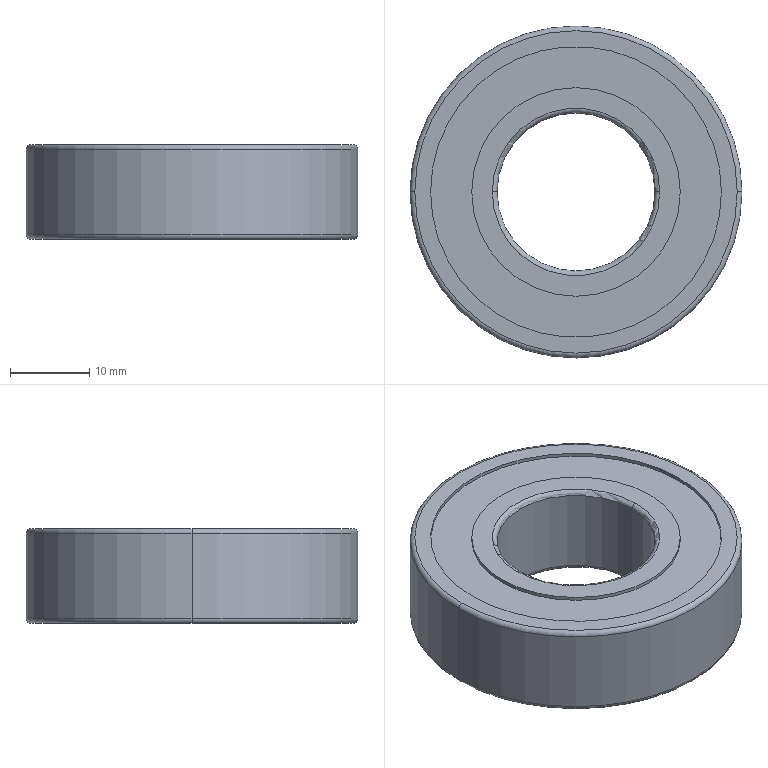Component | SolidWorks | Q1-A12-S21-Q1A.SLDASQ-1_Q1-BGSBB6004ZZ-40.sldasQ-1_Q1-bearing_6004-1 | 1 solid | 26 faces | box 42 x 42 x 12 mm | volume 12378 mm3 | cylinder 12 | torus 8 | plane 6 | commonest cylinder face diameters 26.4 x4 36.8 x4 42 x2 20 x2
build123d program:
from build123d import *


with BuildPart() as part:
    # Sketch1 → Revolve1 (revolve)
    with BuildSketch(Plane.XY, mode=Mode.PRIVATE) as revolve1_sk:
        with BuildLine():
            Line((0.6, 10), (11.4, 10))
            ThreePointArc((11.4, 10), (11.824, 10.176), (12, 10.6))
            Line((12, 10.6), (12, 13.2))
            Line((12, 13.2), (11.567, 13.2))
            Line((11.567, 13.2), (11.567, 18.4))
            Line((11.567, 18.4), (12, 18.4))
            Line((12, 18.4), (12, 20.4))
            ThreePointArc((12, 20.4), (11.824, 20.824), (11.4, 21))
            Line((11.4, 21), (0.6, 21))
            ThreePointArc((0.6, 21), (0.1757, 20.824), (0, 20.4))
            Line((0, 20.4), (0, 18.4))
            Line((0, 18.4), (0.433, 18.4))
            Line((0.433, 18.4), (0.433, 13.2))
            Line((0.433, 13.2), (0, 13.2))
            Line((0, 13.2), (0, 10.6))
            ThreePointArc((0, 10.6), (0.1757, 10.176), (0.6, 10))
        make_face()
    revolve(revolve1_sk.sketch.rotate(Axis((12, 0, 0), (-1, 0, 0)), 270), axis=Axis((12, 0, 0), (-1, 0, 0)))


solid = part.part

# Placed as in the assembly
solid = solid.moved(Location((0, 0, -137.45), (0, 90, 0)))
STEP:
#1=COLOUR_RGB('',0.7922,0.8196,0.9333);
#2=FILL_AREA_STYLE_COLOUR('',#1);
#3=FILL_AREA_STYLE('',(#2));
#4=SURFACE_STYLE_FILL_AREA(#3);
#5=SURFACE_SIDE_STYLE('',(#4));
#6=SURFACE_STYLE_USAGE(.BOTH.,#5);
#7=PRESENTATION_STYLE_ASSIGNMENT((#6));
#8=CARTESIAN_POINT('',(0.5197,0.,-5.867));
#9=VERTEX_POINT('',#8);
#10=CARTESIAN_POINT('',(-0.5197,0.,-5.867));
#11=VERTEX_POINT('',#10);
#12=CARTESIAN_POINT('',(-0.,0.,-5.867));
#13=DIRECTION('',(-0.,0.,-1.));
#14=DIRECTION('',(1.,0.,0.));
#15=AXIS2_PLACEMENT_3D('',#12,#13,#14);
#16=CIRCLE('',#15,0.5197);
#17=EDGE_CURVE('',#9,#11,#16,.T.);
#18=ORIENTED_EDGE('',*,*,#17,.T.);
#19=CARTESIAN_POINT('',(-0.5197,0.,-5.884));
#20=VERTEX_POINT('',#19);
#21=CARTESIAN_POINT('',(-0.5197,0.,-5.411));
#22=DIRECTION('',(-0.,0.,-1.));
#23=VECTOR('',#22,39.37);
#24=LINE('',#21,#23);
#25=EDGE_CURVE('',#11,#20,#24,.T.);
#26=ORIENTED_EDGE('',*,*,#25,.T.);
#27=CARTESIAN_POINT('',(0.5197,0.,-5.884));
#28=VERTEX_POINT('',#27);
#29=CARTESIAN_POINT('',(-0.,0.,-5.884));
#30=DIRECTION('',(-0.,0.,-1.));
#31=DIRECTION('',(1.,0.,0.));
#32=AXIS2_PLACEMENT_3D('',#29,#30,#31);
#33=CIRCLE('',#32,0.5197);
#34=EDGE_CURVE('',#28,#20,#33,.T.);
#35=ORIENTED_EDGE('',*,*,#34,.F.);
#36=CARTESIAN_POINT('',(0.5197,0.,-5.411));
#37=DIRECTION('',(-0.,0.,-1.));
#38=VECTOR('',#37,39.37);
#39=LINE('',#36,#38);
#40=EDGE_CURVE('',#9,#28,#39,.T.);
#41=ORIENTED_EDGE('',*,*,#40,.F.);
#42=EDGE_LOOP('',(#18,#26,#35,#41));
#43=FACE_OUTER_BOUND('',#42,.T.);
#44=CARTESIAN_POINT('',(-0.,0.,-5.411));
#45=DIRECTION('',(-0.,0.,-1.));
#46=DIRECTION('',(1.,0.,0.));
#47=AXIS2_PLACEMENT_3D('',#44,#45,#46);
#48=CYLINDRICAL_SURFACE('',#47,0.5197);
#49=ADVANCED_FACE('',(#43),#48,.T.);
#50=CARTESIAN_POINT('',(-0.7244,-0.,-5.867));
#51=VERTEX_POINT('',#50);
#52=CARTESIAN_POINT('',(0.7244,0.,-5.867));
#53=VERTEX_POINT('',#52);
#54=CARTESIAN_POINT('',(-0.,0.,-5.867));
#55=DIRECTION('',(-0.,0.,-1.));
#56=DIRECTION('',(1.,0.,0.));
#57=AXIS2_PLACEMENT_3D('',#54,#55,#56);
#58=CIRCLE('',#57,0.7244);
#59=EDGE_CURVE('',#51,#53,#58,.T.);
#60=ORIENTED_EDGE('',*,*,#59,.F.);
#61=CARTESIAN_POINT('',(-0.7244,-0.,-5.884));
#62=VERTEX_POINT('',#61);
#63=CARTESIAN_POINT('',(-0.7244,-0.,-5.411));
#64=DIRECTION('',(-0.,0.,-1.));
#65=VECTOR('',#64,39.37);
#66=LINE('',#63,#65);
#67=EDGE_CURVE('',#51,#62,#66,.T.);
#68=ORIENTED_EDGE('',*,*,#67,.T.);
#69=CARTESIAN_POINT('',(0.7244,0.,-5.884));
#70=VERTEX_POINT('',#69);
#71=CARTESIAN_POINT('',(-0.,0.,-5.884));
#72=DIRECTION('',(-0.,0.,-1.));
#73=DIRECTION('',(1.,0.,0.));
#74=AXIS2_PLACEMENT_3D('',#71,#72,#73);
#75=CIRCLE('',#74,0.7244);
#76=EDGE_CURVE('',#62,#70,#75,.T.);
#77=ORIENTED_EDGE('',*,*,#76,.T.);
#78=CARTESIAN_POINT('',(0.7244,0.,-5.411));
#79=DIRECTION('',(-0.,0.,-1.));
#80=VECTOR('',#79,39.37);
#81=LINE('',#78,#80);
#82=EDGE_CURVE('',#53,#70,#81,.T.);
#83=ORIENTED_EDGE('',*,*,#82,.F.);
#84=EDGE_LOOP('',(#60,#68,#77,#83));
#85=FACE_OUTER_BOUND('',#84,.T.);
#86=CARTESIAN_POINT('',(-0.,0.,-5.411));
#87=DIRECTION('',(-0.,0.,-1.));
#88=DIRECTION('',(1.,0.,0.));
#89=AXIS2_PLACEMENT_3D('',#86,#87,#88);
#90=CYLINDRICAL_SURFACE('',#89,0.7244);
#91=ADVANCED_FACE('',(#85),#90,.F.);
#92=CARTESIAN_POINT('',(0.8268,0.,-5.86));
#93=VERTEX_POINT('',#92);
#94=CARTESIAN_POINT('',(-0.8268,-0.,-5.86));
#95=VERTEX_POINT('',#94);
#96=CARTESIAN_POINT('',(-0.,0.,-5.86));
#97=DIRECTION('',(-0.,0.,-1.));
#98=DIRECTION('',(1.,0.,0.));
#99=AXIS2_PLACEMENT_3D('',#96,#97,#98);
#100=CIRCLE('',#99,0.8268);
#101=EDGE_CURVE('',#93,#95,#100,.T.);
#102=ORIENTED_EDGE('',*,*,#101,.T.);
#103=CARTESIAN_POINT('',(-0.8031,-0.,-5.884));
#104=VERTEX_POINT('',#103);
#105=CARTESIAN_POINT('',(-0.8031,-0.,-5.86));
#106=DIRECTION('',(0.,-1.,-0.));
#107=DIRECTION('',(1.,0.,0.));
#108=AXIS2_PLACEMENT_3D('',#105,#106,#107);
#109=CIRCLE('',#108,0.02362);
#110=EDGE_CURVE('',#95,#104,#109,.T.);
#111=ORIENTED_EDGE('',*,*,#110,.T.);
#112=CARTESIAN_POINT('',(0.8031,0.,-5.884));
#113=VERTEX_POINT('',#112);
#114=CARTESIAN_POINT('',(-0.,0.,-5.884));
#115=DIRECTION('',(-0.,0.,-1.));
#116=DIRECTION('',(1.,0.,0.));
#117=AXIS2_PLACEMENT_3D('',#114,#115,#116);
#118=CIRCLE('',#117,0.8031);
#119=EDGE_CURVE('',#113,#104,#118,.T.);
#120=ORIENTED_EDGE('',*,*,#119,.F.);
#121=CARTESIAN_POINT('',(0.8031,0.,-5.86));
#122=DIRECTION('',(-0.,1.,0.));
#123=DIRECTION('',(-1.,-0.,0.));
#124=AXIS2_PLACEMENT_3D('',#121,#122,#123);
#125=CIRCLE('',#124,0.02362);
#126=EDGE_CURVE('',#93,#113,#125,.T.);
#127=ORIENTED_EDGE('',*,*,#126,.F.);
#128=EDGE_LOOP('',(#102,#111,#120,#127));
#129=FACE_OUTER_BOUND('',#128,.T.);
#130=CARTESIAN_POINT('',(-0.,0.,-5.86));
#131=DIRECTION('',(-0.,0.,-1.));
#132=DIRECTION('',(1.,0.,-0.));
#133=AXIS2_PLACEMENT_3D('',#130,#131,#132);
#134=TOROIDAL_SURFACE('',#133,0.8031,0.02362);
#135=ADVANCED_FACE('',(#129),#134,.T.);
#136=CARTESIAN_POINT('',(0.8268,0.,-5.435));
#137=VERTEX_POINT('',#136);
#138=CARTESIAN_POINT('',(-0.8268,-0.,-5.435));
#139=VERTEX_POINT('',#138);
#140=CARTESIAN_POINT('',(-0.,0.,-5.435));
#141=DIRECTION('',(-0.,0.,-1.));
#142=DIRECTION('',(1.,0.,0.));
#143=AXIS2_PLACEMENT_3D('',#140,#141,#142);
#144=CIRCLE('',#143,0.8268);
#145=EDGE_CURVE('',#137,#139,#144,.T.);
#146=ORIENTED_EDGE('',*,*,#145,.T.);
#147=CARTESIAN_POINT('',(-0.8268,-0.,-5.411));
#148=DIRECTION('',(-0.,0.,-1.));
#149=VECTOR('',#148,39.37);
#150=LINE('',#147,#149);
#151=EDGE_CURVE('',#139,#95,#150,.T.);
#152=ORIENTED_EDGE('',*,*,#151,.T.);
#153=ORIENTED_EDGE('',*,*,#101,.F.);
#154=CARTESIAN_POINT('',(0.8268,0.,-5.411));
#155=DIRECTION('',(-0.,0.,-1.));
#156=VECTOR('',#155,39.37);
#157=LINE('',#154,#156);
#158=EDGE_CURVE('',#137,#93,#157,.T.);
#159=ORIENTED_EDGE('',*,*,#158,.F.);
#160=EDGE_LOOP('',(#146,#152,#153,#159));
#161=FACE_OUTER_BOUND('',#160,.T.);
#162=CARTESIAN_POINT('',(-0.,0.,-5.411));
#163=DIRECTION('',(-0.,0.,-1.));
#164=DIRECTION('',(1.,0.,0.));
#165=AXIS2_PLACEMENT_3D('',#162,#163,#164);
#166=CYLINDRICAL_SURFACE('',#165,0.8268);
#167=ADVANCED_FACE('',(#161),#166,.T.);
#168=CARTESIAN_POINT('',(0.8031,0.,-5.411));
#169=VERTEX_POINT('',#168);
#170=CARTESIAN_POINT('',(-0.8031,-0.,-5.411));
#171=VERTEX_POINT('',#170);
#172=CARTESIAN_POINT('',(-0.,0.,-5.411));
#173=DIRECTION('',(-0.,0.,-1.));
#174=DIRECTION('',(1.,0.,0.));
#175=AXIS2_PLACEMENT_3D('',#172,#173,#174);
#176=CIRCLE('',#175,0.8031);
#177=EDGE_CURVE('',#169,#171,#176,.T.);
#178=ORIENTED_EDGE('',*,*,#177,.T.);
#179=CARTESIAN_POINT('',(-0.8031,-0.,-5.435));
#180=DIRECTION('',(0.,-1.,-0.));
#181=DIRECTION('',(1.,0.,0.));
#182=AXIS2_PLACEMENT_3D('',#179,#180,#181);
#183=CIRCLE('',#182,0.02362);
#184=EDGE_CURVE('',#171,#139,#183,.T.);
#185=ORIENTED_EDGE('',*,*,#184,.T.);
#186=ORIENTED_EDGE('',*,*,#145,.F.);
#187=CARTESIAN_POINT('',(0.8031,0.,-5.435));
#188=DIRECTION('',(-0.,1.,0.));
#189=DIRECTION('',(-1.,-0.,0.));
#190=AXIS2_PLACEMENT_3D('',#187,#188,#189);
#191=CIRCLE('',#190,0.02362);
#192=EDGE_CURVE('',#169,#137,#191,.T.);
#193=ORIENTED_EDGE('',*,*,#192,.F.);
#194=EDGE_LOOP('',(#178,#185,#186,#193));
#195=FACE_OUTER_BOUND('',#194,.T.);
#196=CARTESIAN_POINT('',(-0.,0.,-5.435));
#197=DIRECTION('',(-0.,0.,-1.));
#198=DIRECTION('',(1.,0.,-0.));
#199=AXIS2_PLACEMENT_3D('',#196,#197,#198);
#200=TOROIDAL_SURFACE('',#199,0.8031,0.02362);
#201=ADVANCED_FACE('',(#195),#200,.T.);
#202=CARTESIAN_POINT('',(-0.7244,-0.,-5.411));
#203=VERTEX_POINT('',#202);
#204=CARTESIAN_POINT('',(0.7244,0.,-5.411));
#205=VERTEX_POINT('',#204);
#206=CARTESIAN_POINT('',(-0.,0.,-5.411));
#207=DIRECTION('',(-0.,0.,-1.));
#208=DIRECTION('',(1.,0.,0.));
#209=AXIS2_PLACEMENT_3D('',#206,#207,#208);
#210=CIRCLE('',#209,0.7244);
#211=EDGE_CURVE('',#203,#205,#210,.T.);
#212=ORIENTED_EDGE('',*,*,#211,.F.);
#213=CARTESIAN_POINT('',(-0.7244,-0.,-5.428));
#214=VERTEX_POINT('',#213);
#215=CARTESIAN_POINT('',(-0.7244,-0.,-5.411));
#216=DIRECTION('',(-0.,0.,-1.));
#217=VECTOR('',#216,39.37);
#218=LINE('',#215,#217);
#219=EDGE_CURVE('',#203,#214,#218,.T.);
#220=ORIENTED_EDGE('',*,*,#219,.T.);
#221=CARTESIAN_POINT('',(0.7244,0.,-5.428));
#222=VERTEX_POINT('',#221);
#223=CARTESIAN_POINT('',(-0.,0.,-5.428));
#224=DIRECTION('',(-0.,0.,-1.));
#225=DIRECTION('',(1.,0.,0.));
#226=AXIS2_PLACEMENT_3D('',#223,#224,#225);
#227=CIRCLE('',#226,0.7244);
#228=EDGE_CURVE('',#214,#222,#227,.T.);
#229=ORIENTED_EDGE('',*,*,#228,.T.);
#230=CARTESIAN_POINT('',(0.7244,0.,-5.411));
#231=DIRECTION('',(-0.,0.,-1.));
#232=VECTOR('',#231,39.37);
#233=LINE('',#230,#232);
#234=EDGE_CURVE('',#205,#222,#233,.T.);
#235=ORIENTED_EDGE('',*,*,#234,.F.);
#236=EDGE_LOOP('',(#212,#220,#229,#235));
#237=FACE_OUTER_BOUND('',#236,.T.);
#238=CARTESIAN_POINT('',(-0.,0.,-5.411));
#239=DIRECTION('',(-0.,0.,-1.));
#240=DIRECTION('',(1.,0.,0.));
#241=AXIS2_PLACEMENT_3D('',#238,#239,#240);
#242=CYLINDRICAL_SURFACE('',#241,0.7244);
#243=ADVANCED_FACE('',(#237),#242,.F.);
#244=CARTESIAN_POINT('',(0.5197,0.,-5.411));
#245=VERTEX_POINT('',#244);
#246=CARTESIAN_POINT('',(-0.5197,0.,-5.411));
#247=VERTEX_POINT('',#246);
#248=CARTESIAN_POINT('',(-0.,0.,-5.411));
#249=DIRECTION('',(-0.,0.,-1.));
#250=DIRECTION('',(1.,0.,0.));
#251=AXIS2_PLACEMENT_3D('',#248,#249,#250);
#252=CIRCLE('',#251,0.5197);
#253=EDGE_CURVE('',#245,#247,#252,.T.);
#254=ORIENTED_EDGE('',*,*,#253,.T.);
#255=CARTESIAN_POINT('',(-0.5197,0.,-5.428));
#256=VERTEX_POINT('',#255);
#257=CARTESIAN_POINT('',(-0.5197,0.,-5.411));
#258=DIRECTION('',(-0.,0.,-1.));
#259=VECTOR('',#258,39.37);
#260=LINE('',#257,#259);
#261=EDGE_CURVE('',#247,#256,#260,.T.);
#262=ORIENTED_EDGE('',*,*,#261,.T.);
#263=CARTESIAN_POINT('',(0.5197,0.,-5.428));
#264=VERTEX_POINT('',#263);
#265=CARTESIAN_POINT('',(-0.,0.,-5.428));
#266=DIRECTION('',(-0.,0.,-1.));
#267=DIRECTION('',(1.,0.,0.));
#268=AXIS2_PLACEMENT_3D('',#265,#266,#267);
#269=CIRCLE('',#268,0.5197);
#270=EDGE_CURVE('',#264,#256,#269,.T.);
#271=ORIENTED_EDGE('',*,*,#270,.F.);
#272=CARTESIAN_POINT('',(0.5197,0.,-5.411));
#273=DIRECTION('',(-0.,0.,-1.));
#274=VECTOR('',#273,39.37);
#275=LINE('',#272,#274);
#276=EDGE_CURVE('',#245,#264,#275,.T.);
#277=ORIENTED_EDGE('',*,*,#276,.F.);
#278=EDGE_LOOP('',(#254,#262,#271,#277));
#279=FACE_OUTER_BOUND('',#278,.T.);
#280=CARTESIAN_POINT('',(-0.,0.,-5.411));
#281=DIRECTION('',(-0.,0.,-1.));
#282=DIRECTION('',(1.,0.,0.));
#283=AXIS2_PLACEMENT_3D('',#280,#281,#282);
#284=CYLINDRICAL_SURFACE('',#283,0.5197);
#285=ADVANCED_FACE('',(#279),#284,.T.);
#286=CARTESIAN_POINT('',(0.3937,0.,-5.435));
#287=VERTEX_POINT('',#286);
#288=CARTESIAN_POINT('',(-0.3937,0.,-5.435));
#289=VERTEX_POINT('',#288);
#290=CARTESIAN_POINT('',(-0.,0.,-5.435));
#291=DIRECTION('',(-0.,0.,-1.));
#292=DIRECTION('',(1.,0.,0.));
#293=AXIS2_PLACEMENT_3D('',#290,#291,#292);
#294=CIRCLE('',#293,0.3937);
#295=EDGE_CURVE('',#287,#289,#294,.T.);
#296=ORIENTED_EDGE('',*,*,#295,.T.);
#297=CARTESIAN_POINT('',(-0.4173,0.,-5.411));
#298=VERTEX_POINT('',#297);
#299=CARTESIAN_POINT('',(-0.4173,0.,-5.435));
#300=DIRECTION('',(0.,-1.,-0.));
#301=DIRECTION('',(1.,0.,0.));
#302=AXIS2_PLACEMENT_3D('',#299,#300,#301);
#303=CIRCLE('',#302,0.02362);
#304=EDGE_CURVE('',#289,#298,#303,.T.);
#305=ORIENTED_EDGE('',*,*,#304,.T.);
#306=CARTESIAN_POINT('',(0.4173,0.,-5.411));
#307=VERTEX_POINT('',#306);
#308=CARTESIAN_POINT('',(-0.,0.,-5.411));
#309=DIRECTION('',(-0.,0.,-1.));
#310=DIRECTION('',(1.,0.,0.));
#311=AXIS2_PLACEMENT_3D('',#308,#309,#310);
#312=CIRCLE('',#311,0.4173);
#313=EDGE_CURVE('',#307,#298,#312,.T.);
#314=ORIENTED_EDGE('',*,*,#313,.F.);
#315=CARTESIAN_POINT('',(0.4173,0.,-5.435));
#316=DIRECTION('',(-0.,1.,0.));
#317=DIRECTION('',(-1.,-0.,0.));
#318=AXIS2_PLACEMENT_3D('',#315,#316,#317);
#319=CIRCLE('',#318,0.02362);
#320=EDGE_CURVE('',#287,#307,#319,.T.);
#321=ORIENTED_EDGE('',*,*,#320,.F.);
#322=EDGE_LOOP('',(#296,#305,#314,#321));
#323=FACE_OUTER_BOUND('',#322,.T.);
#324=CARTESIAN_POINT('',(-0.,0.,-5.435));
#325=DIRECTION('',(-0.,0.,-1.));
#326=DIRECTION('',(1.,0.,-0.));
#327=AXIS2_PLACEMENT_3D('',#324,#325,#326);
#328=TOROIDAL_SURFACE('',#327,0.4173,0.02362);
#329=ADVANCED_FACE('',(#323),#328,.T.);
#330=CARTESIAN_POINT('',(-0.,0.,-5.435));
#331=DIRECTION('',(-0.,0.,-1.));
#332=DIRECTION('',(1.,0.,0.));
#333=AXIS2_PLACEMENT_3D('',#330,#331,#332);
#334=CIRCLE('',#333,0.3937);
#335=EDGE_CURVE('',#289,#287,#334,.T.);
#336=ORIENTED_EDGE('',*,*,#335,.F.);
#337=CARTESIAN_POINT('',(-0.3937,0.,-5.86));
#338=VERTEX_POINT('',#337);
#339=CARTESIAN_POINT('',(-0.3937,0.,-5.411));
#340=DIRECTION('',(-0.,0.,-1.));
#341=VECTOR('',#340,39.37);
#342=LINE('',#339,#341);
#343=EDGE_CURVE('',#289,#338,#342,.T.);
#344=ORIENTED_EDGE('',*,*,#343,.T.);
#345=CARTESIAN_POINT('',(0.3937,0.,-5.86));
#346=VERTEX_POINT('',#345);
#347=CARTESIAN_POINT('',(-0.,0.,-5.86));
#348=DIRECTION('',(-0.,0.,-1.));
#349=DIRECTION('',(1.,0.,0.));
#350=AXIS2_PLACEMENT_3D('',#347,#348,#349);
#351=CIRCLE('',#350,0.3937);
#352=EDGE_CURVE('',#338,#346,#351,.T.);
#353=ORIENTED_EDGE('',*,*,#352,.T.);
#354=CARTESIAN_POINT('',(0.3937,0.,-5.411));
#355=DIRECTION('',(-0.,0.,-1.));
#356=VECTOR('',#355,39.37);
#357=LINE('',#354,#356);
#358=EDGE_CURVE('',#287,#346,#357,.T.);
#359=ORIENTED_EDGE('',*,*,#358,.F.);
#360=EDGE_LOOP('',(#336,#344,#353,#359));
#361=FACE_OUTER_BOUND('',#360,.T.);
#362=CARTESIAN_POINT('',(-0.,0.,-5.411));
#363=DIRECTION('',(-0.,0.,-1.));
#364=DIRECTION('',(1.,0.,0.));
#365=AXIS2_PLACEMENT_3D('',#362,#363,#364);
#366=CYLINDRICAL_SURFACE('',#365,0.3937);
#367=ADVANCED_FACE('',(#361),#366,.F.);
#368=CARTESIAN_POINT('',(0.4173,0.,-5.884));
#369=VERTEX_POINT('',#368);
#370=CARTESIAN_POINT('',(-0.4173,0.,-5.884));
#371=VERTEX_POINT('',#370);
#372=CARTESIAN_POINT('',(-0.,0.,-5.884));
#373=DIRECTION('',(-0.,0.,-1.));
#374=DIRECTION('',(1.,0.,0.));
#375=AXIS2_PLACEMENT_3D('',#372,#373,#374);
#376=CIRCLE('',#375,0.4173);
#377=EDGE_CURVE('',#369,#371,#376,.T.);
#378=ORIENTED_EDGE('',*,*,#377,.T.);
#379=CARTESIAN_POINT('',(-0.4173,0.,-5.86));
#380=DIRECTION('',(0.,-1.,-0.));
#381=DIRECTION('',(1.,0.,0.));
#382=AXIS2_PLACEMENT_3D('',#379,#380,#381);
#383=CIRCLE('',#382,0.02362);
#384=EDGE_CURVE('',#371,#338,#383,.T.);
#385=ORIENTED_EDGE('',*,*,#384,.T.);
#386=CARTESIAN_POINT('',(-0.,0.,-5.86));
#387=DIRECTION('',(-0.,0.,-1.));
#388=DIRECTION('',(1.,0.,0.));
#389=AXIS2_PLACEMENT_3D('',#386,#387,#388);
#390=CIRCLE('',#389,0.3937);
#391=EDGE_CURVE('',#346,#338,#390,.T.);
#392=ORIENTED_EDGE('',*,*,#391,.F.);
#393=CARTESIAN_POINT('',(0.4173,0.,-5.86));
#394=DIRECTION('',(-0.,1.,0.));
#395=DIRECTION('',(-1.,-0.,0.));
#396=AXIS2_PLACEMENT_3D('',#393,#394,#395);
#397=CIRCLE('',#396,0.02362);
#398=EDGE_CURVE('',#369,#346,#397,.T.);
#399=ORIENTED_EDGE('',*,*,#398,.F.);
#400=EDGE_LOOP('',(#378,#385,#392,#399));
#401=FACE_OUTER_BOUND('',#400,.T.);
#402=CARTESIAN_POINT('',(-0.,0.,-5.86));
#403=DIRECTION('',(-0.,0.,-1.));
#404=DIRECTION('',(1.,0.,-0.));
#405=AXIS2_PLACEMENT_3D('',#402,#403,#404);
#406=TOROIDAL_SURFACE('',#405,0.4173,0.02362);
#407=ADVANCED_FACE('',(#401),#406,.T.);
#408=ORIENTED_EDGE('',*,*,#384,.F.);
#409=CARTESIAN_POINT('',(-0.,0.,-5.884));
#410=DIRECTION('',(-0.,0.,-1.));
#411=DIRECTION('',(1.,0.,0.));
#412=AXIS2_PLACEMENT_3D('',#409,#410,#411);
#413=CIRCLE('',#412,0.4173);
#414=EDGE_CURVE('',#371,#369,#413,.T.);
#415=ORIENTED_EDGE('',*,*,#414,.T.);
#416=ORIENTED_EDGE('',*,*,#398,.T.);
#417=ORIENTED_EDGE('',*,*,#352,.F.);
#418=EDGE_LOOP('',(#408,#415,#416,#417));
#419=FACE_OUTER_BOUND('',#418,.T.);
#420=CARTESIAN_POINT('',(-0.,0.,-5.86));
#421=DIRECTION('',(-0.,0.,-1.));
#422=DIRECTION('',(1.,0.,-0.));
#423=AXIS2_PLACEMENT_3D('',#420,#421,#422);
#424=TOROIDAL_SURFACE('',#423,0.4173,0.02362);
#425=ADVANCED_FACE('',(#419),#424,.T.);
#426=ORIENTED_EDGE('',*,*,#343,.F.);
#427=ORIENTED_EDGE('',*,*,#295,.F.);
#428=ORIENTED_EDGE('',*,*,#358,.T.);
#429=ORIENTED_EDGE('',*,*,#391,.T.);
#430=EDGE_LOOP('',(#426,#427,#428,#429));
#431=FACE_OUTER_BOUND('',#430,.T.);
#432=CARTESIAN_POINT('',(-0.,0.,-5.411));
#433=DIRECTION('',(-0.,0.,-1.));
#434=DIRECTION('',(1.,0.,0.));
#435=AXIS2_PLACEMENT_3D('',#432,#433,#434);
#436=CYLINDRICAL_SURFACE('',#435,0.3937);
#437=ADVANCED_FACE('',(#431),#436,.F.);
#438=ORIENTED_EDGE('',*,*,#304,.F.);
#439=ORIENTED_EDGE('',*,*,#335,.T.);
#440=ORIENTED_EDGE('',*,*,#320,.T.);
#441=CARTESIAN_POINT('',(-0.,0.,-5.411));
#442=DIRECTION('',(-0.,0.,-1.));
#443=DIRECTION('',(1.,0.,0.));
#444=AXIS2_PLACEMENT_3D('',#441,#442,#443);
#445=CIRCLE('',#444,0.4173);
#446=EDGE_CURVE('',#298,#307,#445,.T.);
#447=ORIENTED_EDGE('',*,*,#446,.F.);
#448=EDGE_LOOP('',(#438,#439,#440,#447));
#449=FACE_OUTER_BOUND('',#448,.T.);
#450=CARTESIAN_POINT('',(-0.,0.,-5.435));
#451=DIRECTION('',(-0.,0.,-1.));
#452=DIRECTION('',(1.,0.,-0.));
#453=AXIS2_PLACEMENT_3D('',#450,#451,#452);
#454=TOROIDAL_SURFACE('',#453,0.4173,0.02362);
#455=ADVANCED_FACE('',(#449),#454,.T.);
#456=ORIENTED_EDGE('',*,*,#253,.F.);
#457=CARTESIAN_POINT('',(-0.,0.,-5.411));
#458=DIRECTION('',(-0.,0.,-1.));
#459=DIRECTION('',(1.,0.,0.));
#460=AXIS2_PLACEMENT_3D('',#457,#458,#459);
#461=CIRCLE('',#460,0.5197);
#462=EDGE_CURVE('',#247,#245,#461,.T.);
#463=ORIENTED_EDGE('',*,*,#462,.F.);
#464=EDGE_LOOP('',(#456,#463));
#465=FACE_OUTER_BOUND('',#464,.T.);
#466=ORIENTED_EDGE('',*,*,#313,.T.);
#467=ORIENTED_EDGE('',*,*,#446,.T.);
#468=EDGE_LOOP('',(#466,#467));
#469=FACE_BOUND('',#468,.T.);
#470=CARTESIAN_POINT('',(-0.,-0.4173,-5.411));
#471=DIRECTION('',(0.,0.,-1.));
#472=DIRECTION('',(1.,0.,0.));
#473=AXIS2_PLACEMENT_3D('',#470,#471,#472);
#474=PLANE('',#473);
#475=ADVANCED_FACE('',(#465,#469),#474,.F.);
#476=ORIENTED_EDGE('',*,*,#261,.F.);
#477=ORIENTED_EDGE('',*,*,#462,.T.);
#478=ORIENTED_EDGE('',*,*,#276,.T.);
#479=CARTESIAN_POINT('',(-0.,0.,-5.428));
#480=DIRECTION('',(-0.,0.,-1.));
#481=DIRECTION('',(1.,0.,0.));
#482=AXIS2_PLACEMENT_3D('',#479,#480,#481);
#483=CIRCLE('',#482,0.5197);
#484=EDGE_CURVE('',#256,#264,#483,.T.);
#485=ORIENTED_EDGE('',*,*,#484,.F.);
#486=EDGE_LOOP('',(#476,#477,#478,#485));
#487=FACE_OUTER_BOUND('',#486,.T.);
#488=CARTESIAN_POINT('',(-0.,0.,-5.411));
#489=DIRECTION('',(-0.,0.,-1.));
#490=DIRECTION('',(1.,0.,0.));
#491=AXIS2_PLACEMENT_3D('',#488,#489,#490);
#492=CYLINDRICAL_SURFACE('',#491,0.5197);
#493=ADVANCED_FACE('',(#487),#492,.T.);
#494=CARTESIAN_POINT('',(-0.,0.,-5.428));
#495=DIRECTION('',(-0.,0.,-1.));
#496=DIRECTION('',(1.,0.,0.));
#497=AXIS2_PLACEMENT_3D('',#494,#495,#496);
#498=CIRCLE('',#497,0.7244);
#499=EDGE_CURVE('',#222,#214,#498,.T.);
#500=ORIENTED_EDGE('',*,*,#499,.F.);
#501=ORIENTED_EDGE('',*,*,#228,.F.);
#502=EDGE_LOOP('',(#500,#501));
#503=FACE_OUTER_BOUND('',#502,.T.);
#504=ORIENTED_EDGE('',*,*,#270,.T.);
#505=ORIENTED_EDGE('',*,*,#484,.T.);
#506=EDGE_LOOP('',(#504,#505));
#507=FACE_BOUND('',#506,.T.);
#508=CARTESIAN_POINT('',(-0.,-0.5197,-5.428));
#509=DIRECTION('',(0.,0.,-1.));
#510=DIRECTION('',(1.,0.,0.));
#511=AXIS2_PLACEMENT_3D('',#508,#509,#510);
#512=PLANE('',#511);
#513=ADVANCED_FACE('',(#503,#507),#512,.F.);
#514=ORIENTED_EDGE('',*,*,#219,.F.);
#515=CARTESIAN_POINT('',(-0.,0.,-5.411));
#516=DIRECTION('',(-0.,0.,-1.));
#517=DIRECTION('',(1.,0.,0.));
#518=AXIS2_PLACEMENT_3D('',#515,#516,#517);
#519=CIRCLE('',#518,0.7244);
#520=EDGE_CURVE('',#205,#203,#519,.T.);
#521=ORIENTED_EDGE('',*,*,#520,.F.);
#522=ORIENTED_EDGE('',*,*,#234,.T.);
#523=ORIENTED_EDGE('',*,*,#499,.T.);
#524=EDGE_LOOP('',(#514,#521,#522,#523));
#525=FACE_OUTER_BOUND('',#524,.T.);
#526=CARTESIAN_POINT('',(-0.,0.,-5.411));
#527=DIRECTION('',(-0.,0.,-1.));
#528=DIRECTION('',(1.,0.,0.));
#529=AXIS2_PLACEMENT_3D('',#526,#527,#528);
#530=CYLINDRICAL_SURFACE('',#529,0.7244);
#531=ADVANCED_FACE('',(#525),#530,.F.);
#532=ORIENTED_EDGE('',*,*,#177,.F.);
#533=CARTESIAN_POINT('',(-0.,0.,-5.411));
#534=DIRECTION('',(-0.,0.,-1.));
#535=DIRECTION('',(1.,0.,0.));
#536=AXIS2_PLACEMENT_3D('',#533,#534,#535);
#537=CIRCLE('',#536,0.8031);
#538=EDGE_CURVE('',#171,#169,#537,.T.);
#539=ORIENTED_EDGE('',*,*,#538,.F.);
#540=EDGE_LOOP('',(#532,#539));
#541=FACE_OUTER_BOUND('',#540,.T.);
#542=ORIENTED_EDGE('',*,*,#520,.T.);
#543=ORIENTED_EDGE('',*,*,#211,.T.);
#544=EDGE_LOOP('',(#542,#543));
#545=FACE_BOUND('',#544,.T.);
#546=CARTESIAN_POINT('',(-0.,-0.7244,-5.411));
#547=DIRECTION('',(0.,0.,-1.));
#548=DIRECTION('',(1.,0.,0.));
#549=AXIS2_PLACEMENT_3D('',#546,#547,#548);
#550=PLANE('',#549);
#551=ADVANCED_FACE('',(#541,#545),#550,.F.);
#552=ORIENTED_EDGE('',*,*,#184,.F.);
#553=ORIENTED_EDGE('',*,*,#538,.T.);
#554=ORIENTED_EDGE('',*,*,#192,.T.);
#555=CARTESIAN_POINT('',(-0.,0.,-5.435));
#556=DIRECTION('',(-0.,0.,-1.));
#557=DIRECTION('',(1.,0.,0.));
#558=AXIS2_PLACEMENT_3D('',#555,#556,#557);
#559=CIRCLE('',#558,0.8268);
#560=EDGE_CURVE('',#139,#137,#559,.T.);
#561=ORIENTED_EDGE('',*,*,#560,.F.);
#562=EDGE_LOOP('',(#552,#553,#554,#561));
#563=FACE_OUTER_BOUND('',#562,.T.);
#564=CARTESIAN_POINT('',(-0.,0.,-5.435));
#565=DIRECTION('',(-0.,0.,-1.));
#566=DIRECTION('',(1.,0.,-0.));
#567=AXIS2_PLACEMENT_3D('',#564,#565,#566);
#568=TOROIDAL_SURFACE('',#567,0.8031,0.02362);
#569=ADVANCED_FACE('',(#563),#568,.T.);
#570=ORIENTED_EDGE('',*,*,#151,.F.);
#571=ORIENTED_EDGE('',*,*,#560,.T.);
#572=ORIENTED_EDGE('',*,*,#158,.T.);
#573=CARTESIAN_POINT('',(-0.,0.,-5.86));
#574=DIRECTION('',(-0.,0.,-1.));
#575=DIRECTION('',(1.,0.,0.));
#576=AXIS2_PLACEMENT_3D('',#573,#574,#575);
#577=CIRCLE('',#576,0.8268);
#578=EDGE_CURVE('',#95,#93,#577,.T.);
#579=ORIENTED_EDGE('',*,*,#578,.F.);
#580=EDGE_LOOP('',(#570,#571,#572,#579));
#581=FACE_OUTER_BOUND('',#580,.T.);
#582=CARTESIAN_POINT('',(-0.,0.,-5.411));
#583=DIRECTION('',(-0.,0.,-1.));
#584=DIRECTION('',(1.,0.,0.));
#585=AXIS2_PLACEMENT_3D('',#582,#583,#584);
#586=CYLINDRICAL_SURFACE('',#585,0.8268);
#587=ADVANCED_FACE('',(#581),#586,.T.);
#588=ORIENTED_EDGE('',*,*,#110,.F.);
#589=ORIENTED_EDGE('',*,*,#578,.T.);
#590=ORIENTED_EDGE('',*,*,#126,.T.);
#591=CARTESIAN_POINT('',(-0.,0.,-5.884));
#592=DIRECTION('',(-0.,0.,-1.));
#593=DIRECTION('',(1.,0.,0.));
#594=AXIS2_PLACEMENT_3D('',#591,#592,#593);
#595=CIRCLE('',#594,0.8031);
#596=EDGE_CURVE('',#104,#113,#595,.T.);
#597=ORIENTED_EDGE('',*,*,#596,.F.);
#598=EDGE_LOOP('',(#588,#589,#590,#597));
#599=FACE_OUTER_BOUND('',#598,.T.);
#600=CARTESIAN_POINT('',(-0.,0.,-5.86));
#601=DIRECTION('',(-0.,0.,-1.));
#602=DIRECTION('',(1.,0.,-0.));
#603=AXIS2_PLACEMENT_3D('',#600,#601,#602);
#604=TOROIDAL_SURFACE('',#603,0.8031,0.02362);
#605=ADVANCED_FACE('',(#599),#604,.T.);
#606=CARTESIAN_POINT('',(-0.,0.,-5.884));
#607=DIRECTION('',(-0.,0.,-1.));
#608=DIRECTION('',(1.,0.,0.));
#609=AXIS2_PLACEMENT_3D('',#606,#607,#608);
#610=CIRCLE('',#609,0.7244);
#611=EDGE_CURVE('',#70,#62,#610,.T.);
#612=ORIENTED_EDGE('',*,*,#611,.F.);
#613=ORIENTED_EDGE('',*,*,#76,.F.);
#614=EDGE_LOOP('',(#612,#613));
#615=FACE_BOUND('',#614,.T.);
#616=ORIENTED_EDGE('',*,*,#119,.T.);
#617=ORIENTED_EDGE('',*,*,#596,.T.);
#618=EDGE_LOOP('',(#616,#617));
#619=FACE_OUTER_BOUND('',#618,.T.);
#620=CARTESIAN_POINT('',(-0.,-0.8031,-5.884));
#621=DIRECTION('',(-0.,-0.,1.));
#622=DIRECTION('',(-1.,-0.,-0.));
#623=AXIS2_PLACEMENT_3D('',#620,#621,#622);
#624=PLANE('',#623);
#625=ADVANCED_FACE('',(#615,#619),#624,.F.);
#626=ORIENTED_EDGE('',*,*,#67,.F.);
#627=CARTESIAN_POINT('',(-0.,0.,-5.867));
#628=DIRECTION('',(-0.,0.,-1.));
#629=DIRECTION('',(1.,0.,0.));
#630=AXIS2_PLACEMENT_3D('',#627,#628,#629);
#631=CIRCLE('',#630,0.7244);
#632=EDGE_CURVE('',#53,#51,#631,.T.);
#633=ORIENTED_EDGE('',*,*,#632,.F.);
#634=ORIENTED_EDGE('',*,*,#82,.T.);
#635=ORIENTED_EDGE('',*,*,#611,.T.);
#636=EDGE_LOOP('',(#626,#633,#634,#635));
#637=FACE_OUTER_BOUND('',#636,.T.);
#638=CARTESIAN_POINT('',(-0.,0.,-5.411));
#639=DIRECTION('',(-0.,0.,-1.));
#640=DIRECTION('',(1.,0.,0.));
#641=AXIS2_PLACEMENT_3D('',#638,#639,#640);
#642=CYLINDRICAL_SURFACE('',#641,0.7244);
#643=ADVANCED_FACE('',(#637),#642,.F.);
#644=ORIENTED_EDGE('',*,*,#17,.F.);
#645=CARTESIAN_POINT('',(-0.,0.,-5.867));
#646=DIRECTION('',(-0.,0.,-1.));
#647=DIRECTION('',(1.,0.,0.));
#648=AXIS2_PLACEMENT_3D('',#645,#646,#647);
#649=CIRCLE('',#648,0.5197);
#650=EDGE_CURVE('',#11,#9,#649,.T.);
#651=ORIENTED_EDGE('',*,*,#650,.F.);
#652=EDGE_LOOP('',(#644,#651));
#653=FACE_BOUND('',#652,.T.);
#654=ORIENTED_EDGE('',*,*,#632,.T.);
#655=ORIENTED_EDGE('',*,*,#59,.T.);
#656=EDGE_LOOP('',(#654,#655));
#657=FACE_OUTER_BOUND('',#656,.T.);
#658=CARTESIAN_POINT('',(-0.,-0.7244,-5.867));
#659=DIRECTION('',(-0.,-0.,1.));
#660=DIRECTION('',(-1.,-0.,-0.));
#661=AXIS2_PLACEMENT_3D('',#658,#659,#660);
#662=PLANE('',#661);
#663=ADVANCED_FACE('',(#653,#657),#662,.F.);
#664=ORIENTED_EDGE('',*,*,#25,.F.);
#665=ORIENTED_EDGE('',*,*,#650,.T.);
#666=ORIENTED_EDGE('',*,*,#40,.T.);
#667=CARTESIAN_POINT('',(-0.,0.,-5.884));
#668=DIRECTION('',(-0.,0.,-1.));
#669=DIRECTION('',(1.,0.,0.));
#670=AXIS2_PLACEMENT_3D('',#667,#668,#669);
#671=CIRCLE('',#670,0.5197);
#672=EDGE_CURVE('',#20,#28,#671,.T.);
#673=ORIENTED_EDGE('',*,*,#672,.F.);
#674=EDGE_LOOP('',(#664,#665,#666,#673));
#675=FACE_OUTER_BOUND('',#674,.T.);
#676=CARTESIAN_POINT('',(-0.,0.,-5.411));
#677=DIRECTION('',(-0.,0.,-1.));
#678=DIRECTION('',(1.,0.,0.));
#679=AXIS2_PLACEMENT_3D('',#676,#677,#678);
#680=CYLINDRICAL_SURFACE('',#679,0.5197);
#681=ADVANCED_FACE('',(#675),#680,.T.);
#682=ORIENTED_EDGE('',*,*,#377,.F.);
#683=ORIENTED_EDGE('',*,*,#414,.F.);
#684=EDGE_LOOP('',(#682,#683));
#685=FACE_BOUND('',#684,.T.);
#686=ORIENTED_EDGE('',*,*,#34,.T.);
#687=ORIENTED_EDGE('',*,*,#672,.T.);
#688=EDGE_LOOP('',(#686,#687));
#689=FACE_OUTER_BOUND('',#688,.T.);
#690=CARTESIAN_POINT('',(-0.,-0.5197,-5.884));
#691=DIRECTION('',(-0.,-0.,1.));
#692=DIRECTION('',(-1.,-0.,-0.));
#693=AXIS2_PLACEMENT_3D('',#690,#691,#692);
#694=PLANE('',#693);
#695=ADVANCED_FACE('',(#685,#689),#694,.F.);
#696=CLOSED_SHELL('',(#49,#91,#135,#167,#201,#243,#285,#329,#367,#407,#425,#437,#455,#475,#493,#513,#531,#551,#569,#587,#605,#625,#643,#663,#681,#695));
#697=MANIFOLD_SOLID_BREP('',#696);
#698=STYLED_ITEM('',(#7),#697);
#699=(LENGTH_UNIT()NAMED_UNIT(*)SI_UNIT($,.METRE.));
#700=LENGTH_MEASURE_WITH_UNIT(LENGTH_MEASURE(0.0254),#699);
#701=DIMENSIONAL_EXPONENTS(1.,0.,0.,0.,0.,0.,0.);
#702=(CONVERSION_BASED_UNIT('',#700)LENGTH_UNIT()NAMED_UNIT(#701));
#703=UNCERTAINTY_MEASURE_WITH_UNIT(LENGTH_MEASURE(0.00001),#702,'','');
#704=(NAMED_UNIT(*)PLANE_ANGLE_UNIT()SI_UNIT($,.RADIAN.));
#705=(NAMED_UNIT(*)SI_UNIT($,.STERADIAN.)SOLID_ANGLE_UNIT());
#706=(GEOMETRIC_REPRESENTATION_CONTEXT(3)GLOBAL_UNCERTAINTY_ASSIGNED_CONTEXT((#703))GLOBAL_UNIT_ASSIGNED_CONTEXT((#702,#704,#705))REPRESENTATION_CONTEXT('',''));
#707=MECHANICAL_DESIGN_GEOMETRIC_PRESENTATION_REPRESENTATION('',(#698),#706);
#708=PRESENTATION_LAYER_ASSIGNMENT('','',(#698));
#709=CARTESIAN_POINT('',(0.,0.,0.));
#710=DIRECTION('',(0.,0.,1.));
#711=DIRECTION('',(1.,0.,0.));
#712=AXIS2_PLACEMENT_3D('',#709,#710,#711);
#713=(LENGTH_UNIT()NAMED_UNIT(*)SI_UNIT($,.METRE.));
#714=LENGTH_MEASURE_WITH_UNIT(LENGTH_MEASURE(0.0254),#713);
#715=DIMENSIONAL_EXPONENTS(1.,0.,0.,0.,0.,0.,0.);
#716=(CONVERSION_BASED_UNIT('',#714)LENGTH_UNIT()NAMED_UNIT(#715));
#717=UNCERTAINTY_MEASURE_WITH_UNIT(LENGTH_MEASURE(0.00001),#716,'','');
#718=(NAMED_UNIT(*)PLANE_ANGLE_UNIT()SI_UNIT($,.RADIAN.));
#719=(NAMED_UNIT(*)SI_UNIT($,.STERADIAN.)SOLID_ANGLE_UNIT());
#720=(GEOMETRIC_REPRESENTATION_CONTEXT(3)GLOBAL_UNCERTAINTY_ASSIGNED_CONTEXT((#717))GLOBAL_UNIT_ASSIGNED_CONTEXT((#716,#718,#719))REPRESENTATION_CONTEXT('',''));
#721=ADVANCED_BREP_SHAPE_REPRESENTATION('',(#697,#712),#720);